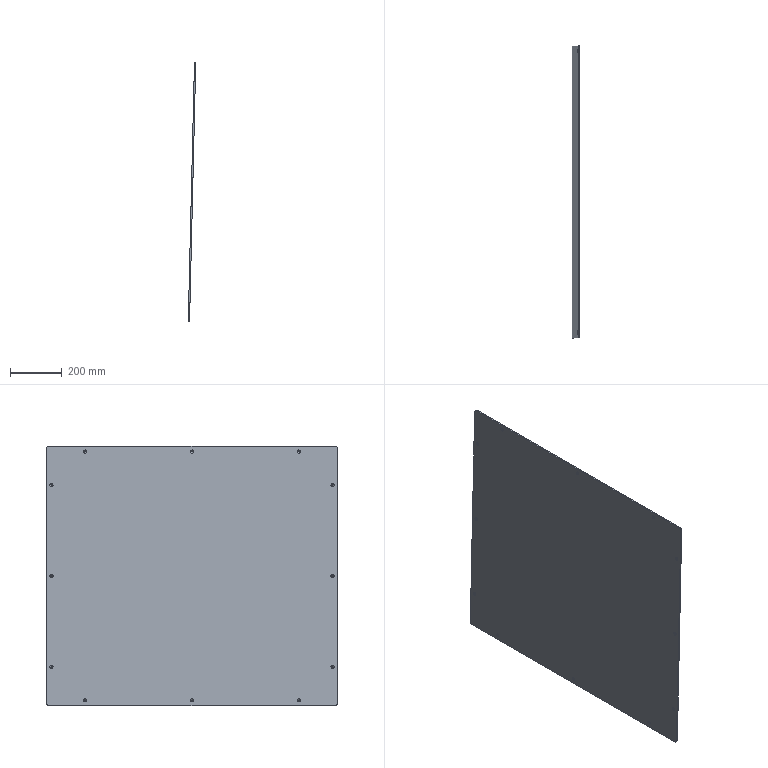Component | SolidWorks | A3020-1 | 1 solid | 58 faces | volume 5621059 mm3 | cylinder 28 | cone 24 | plane 6 | commonest cylinder face diameters 6.6 x24 20 x4 | material PC